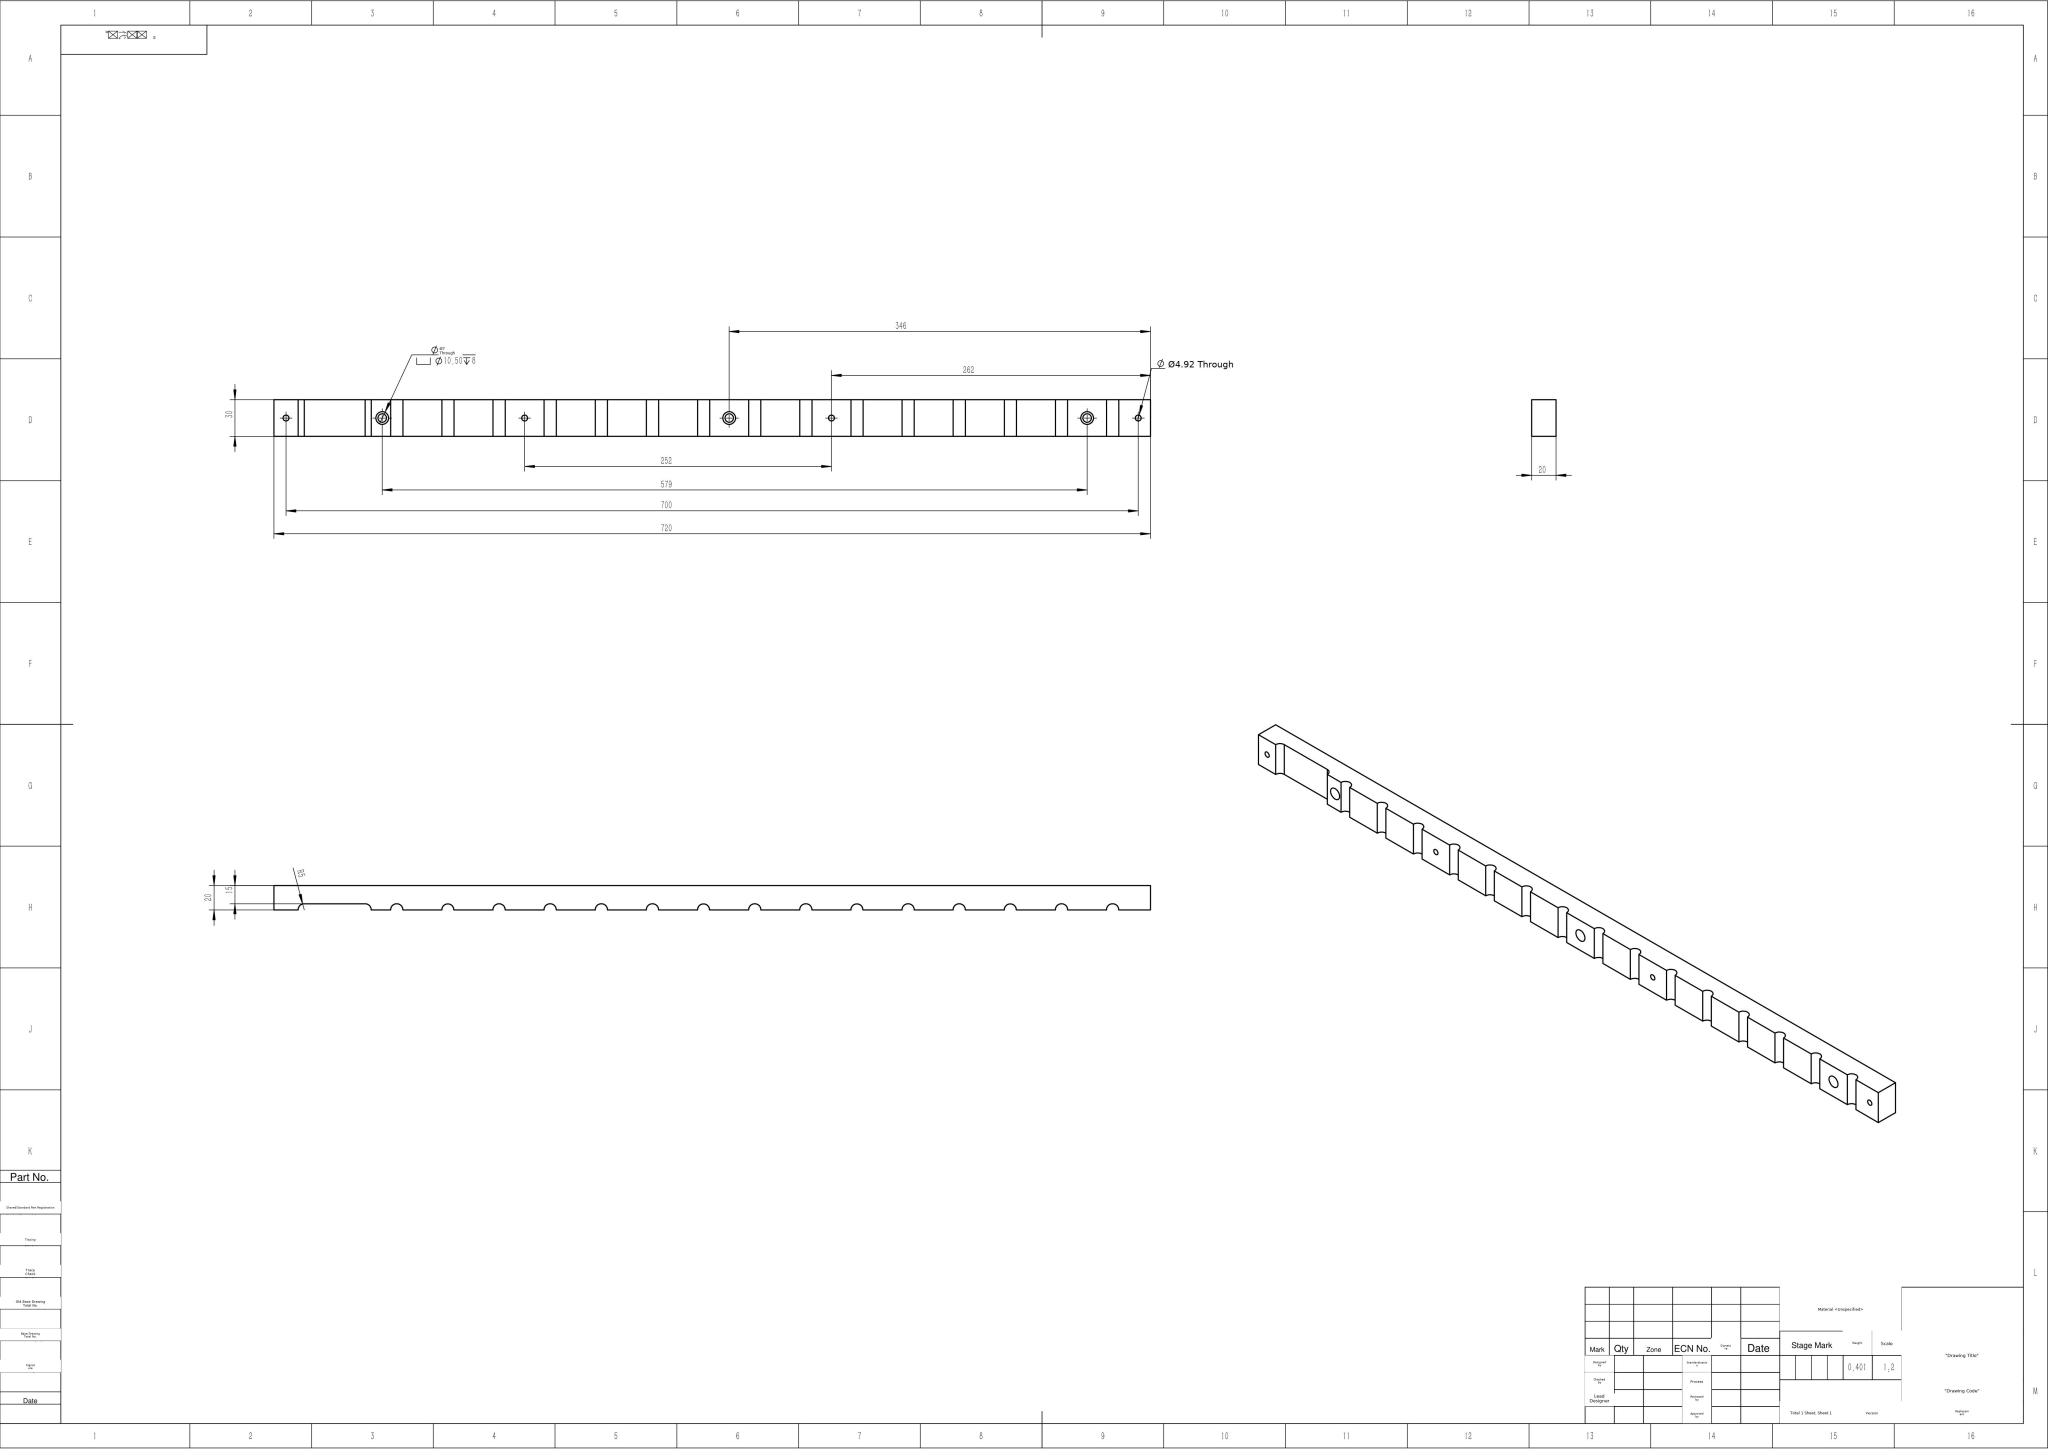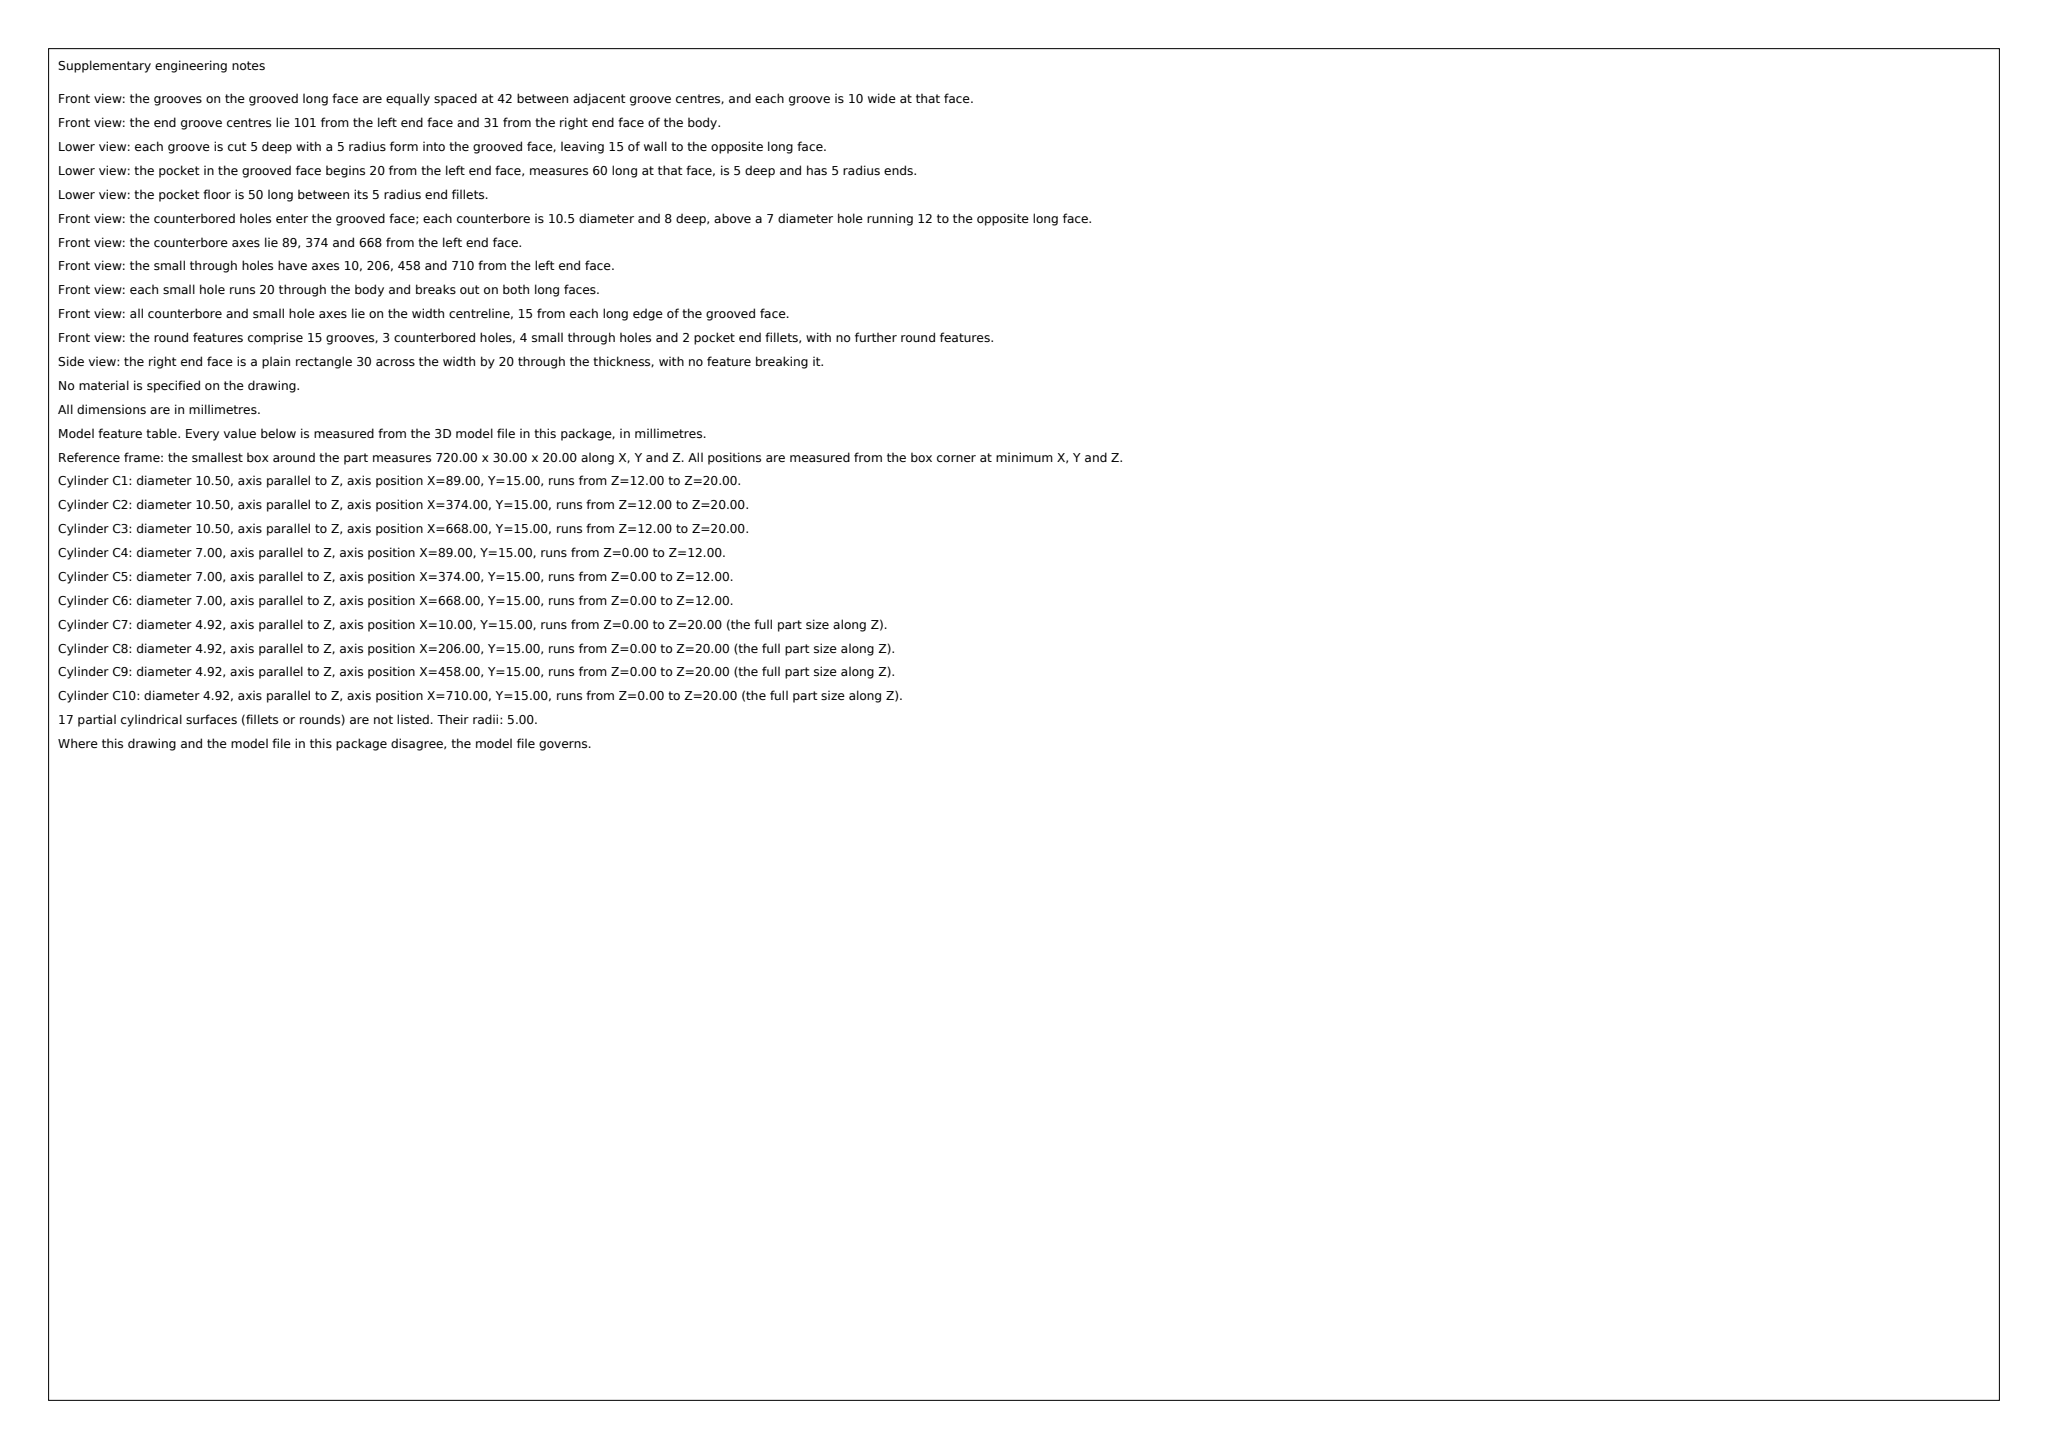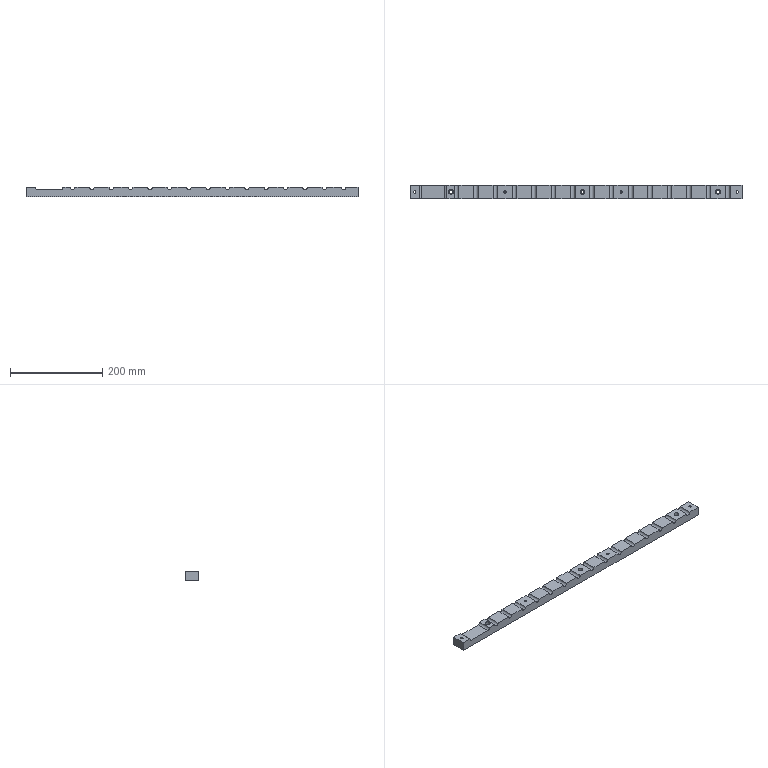Part | SolidWorks | mm | 1 solid | 63 faces | box 720 x 30 x 20 mm | volume 400668 mm3 | cylinder 37 | plane 26 | commonest cylinder face diameters 10 x17 4.917 x8 10.5 x6 7 x6
Drawing notes:
3X Ø7 THRU, CBORE Ø10.50 DP 8 AT 89, 374 & 668 FROM LH END | from the solid: Ø7 z-holes at x=89,374,668, y=15; Ø10.5 cbore 8 deep, same x
17X R5 GROOVE, 10 WIDE, THRU 30 WIDTH, ON TOP FACE Z20 | from the solid: Ø10 y-axis cylinders, len 30, at z=20, 17 instances
R5 GROOVES: 1ST AT 25, 2ND AT 75 FROM LH END | from the solid: groove x-positions 25 and 75 from x=0 face
15X R5 GROOVE EQ SP 42, 101 TO 689 FROM LH END | from the solid: grooves at x=101..689 step 42 (15 off)
4X Ø4.92 THRU 20 AT 10, 206, 458 & 710 FROM LH END | from the solid: Ø4.917 z-holes len 20 (full thk) at x=10,206,458,710, y=15